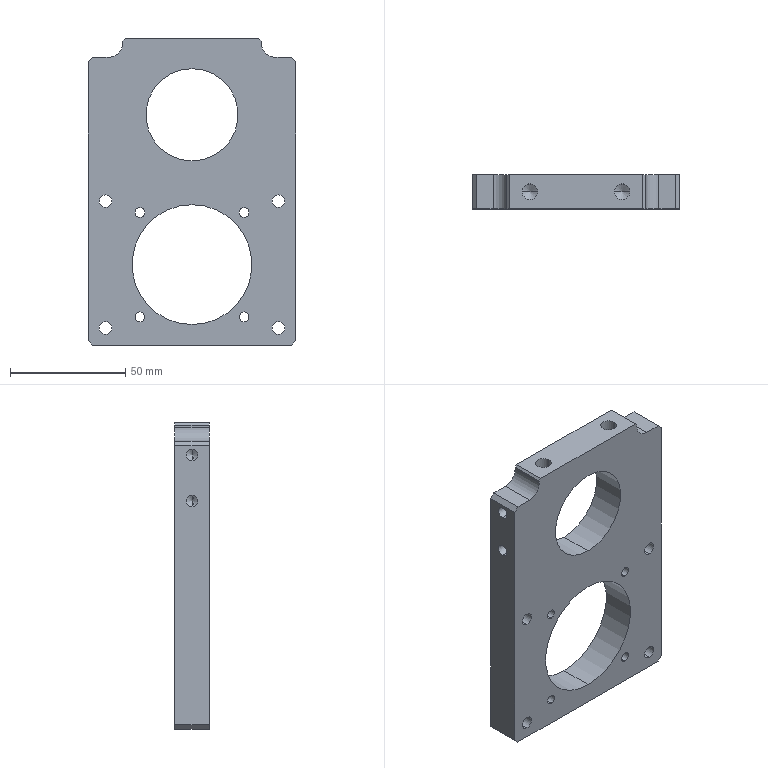Component | SolidWorks | H2020022-0413-1-1 | 1 solid | 74 faces | box 90 x 14.8 x 133 mm | volume 117995 mm3 | cylinder 42 | plane 20 | cone 12 | commonest cylinder face diameters 5 x8 4.2 x8 10 x8 5.5 x8 6.8 x4 40 x2 52 x2 12 x2 | material 6061 Aluminum Alloy
build123d program:
from build123d import *

# Parameters (mm, degrees)
SKETCH1_W                                       = 90
SKETCH1_H                                       = 125
BOSS_EXTRUDE1_DEPTH                             = 14.8
SKETCH4_R                                       = 26
CUT_EXTRUDE1_DEPTH                              = 155.739
M5_HEX_SOCKET_HEAD_CAP_SCREW_CBORE1_D           = 5.5
M5_HEX_SOCKET_HEAD_CAP_SCREW_CBORE1_CBORE_D     = 10
M5_HEX_SOCKET_HEAD_CAP_SCREW_CBORE1_CBORE_DEPTH = 5.4
M6_TAPPED_HOLE1_AT_2_COUNT                      = 2
M6_TAPPED_HOLE1_AT_2_PITCH                      = 20
CHAMFER1_SIZE                                   = 2
M5_TAPPED_HOLE2_D                               = 4.2
CIRPATTERN1_COUNT                               = 4
SKETCH20_R                                      = 20
CUT_EXTRUDE4_DEPTH                              = 155.739
SKETCH21_W                                      = 8
SKETCH21_H                                      = 14.8
BOSS_EXTRUDE2_DEPTH                             = 30
M8_TAPPED_HOLE1_D                               = 6.8
M8_TAPPED_HOLE1_DEPTH                           = 13.75
M8_TAPPED_HOLE1_TIP                             = 2.043
FILLET1_R                                       = 6
CHAMFER2_SIZE                                   = 1


with BuildPart() as part:
    # Sketch1 → Boss-Extrude1 (new body)
    with BuildSketch(Plane(origin=(0, 0, 0), x_dir=(1, 0, 0), z_dir=(0, 1, 0))):
        with Locations((45, 62.5)):
            Rectangle(SKETCH1_W, SKETCH1_H)
    extrude(amount=BOSS_EXTRUDE1_DEPTH)

    # Sketch4 → Cut-Extrude1 (cut, through all)
    with BuildSketch(Plane(origin=(0, 14.8, 0), x_dir=(1, 0, 0), z_dir=(0, 1, 0))):
        with Locations(Location((45, 90, 0), (0, 0, 270))):
            Circle(SKETCH4_R)
    extrude(amount=-CUT_EXTRUDE1_DEPTH, mode=Mode.SUBTRACT)

    # M5 Hex Socket Head Cap Screw CBORE1 (through all)
    with Locations(Plane(origin=(0, 14.8, 0), x_dir=(1, 0, 0), z_dir=(0, 1, 0))):
        with Locations((7.5, 62.5), (82.5, 62.5), (82.5, 117.5), (7.5, 117.5)):
            CounterBoreHole(M5_HEX_SOCKET_HEAD_CAP_SCREW_CBORE1_D / 2, M5_HEX_SOCKET_HEAD_CAP_SCREW_CBORE1_CBORE_D / 2, M5_HEX_SOCKET_HEAD_CAP_SCREW_CBORE1_CBORE_DEPTH)

    # Sketch12 → M6 Tapped Hole1 (revolve, cut)
    with BuildSketch(Plane(origin=(90, 7.4, -6), x_dir=(0, 0, -1), z_dir=(0, 1, 0))):
        Polygon((0, 0), (0, 16.502), (2.5, 15), (2.5, 0), align=None)
    m6_tapped_hole1 = revolve(axis=Axis((96.35, 7.4, -6), (-1, 0, 0)), mode=Mode.SUBTRACT)

    # M6 Tapped Hole1 at 2: M6 Tapped Hole1 ×2
    with Locations(*[(0, 0, -i * M6_TAPPED_HOLE1_AT_2_PITCH) for i in range(1, M6_TAPPED_HOLE1_AT_2_COUNT)]):
        add(m6_tapped_hole1, mode=Mode.SUBTRACT)

    # Chamfer1
    chamfer1_edges = [part.edges().sort_by_distance(p)[0] for p in [
        (0, 7.4, -125),
        (90, 7.4, -125),
        (90, 7.4, 0),
        (0, 7.4, 0),
    ]]
    chamfer(chamfer1_edges, length=CHAMFER1_SIZE)

    # M5 Tapped Hole2 (through all)
    with Locations(Plane(origin=(0, 14.8, 0), x_dir=(1, 0, 0), z_dir=(0, 1, 0))):
        with Locations((22.373, 112.627)):
            m5_tapped_hole2 = Hole(M5_TAPPED_HOLE2_D / 2)

    # CirPattern1: M5 Tapped Hole2 ×4 about axis
    cirpattern1_axis = Axis((45, 0, -90), (0, 1, 0))
    for i in range(1, CIRPATTERN1_COUNT):
        add(m5_tapped_hole2.rotate(cirpattern1_axis, i * 360 / CIRPATTERN1_COUNT), mode=Mode.SUBTRACT)

    # Sketch20 → Cut-Extrude4 (cut, through all)
    with BuildSketch(Plane(origin=(0, 14.8, 0), x_dir=(1, 0, 0), z_dir=(0, 1, 0))):
        with Locations(Location((45, 25, 0), (0, 0, 270))):
            Circle(SKETCH20_R)
    extrude(amount=-CUT_EXTRUDE4_DEPTH, mode=Mode.SUBTRACT)

    # Sketch21 → Boss-Extrude2 (add, symmetric)
    with BuildSketch(Plane(origin=(45, 0, 0), x_dir=(0, 0, -1), z_dir=(1, 0, 0))):
        with Locations((-4, 7.4)):
            Rectangle(SKETCH21_W, SKETCH21_H)
    extrude(amount=BOSS_EXTRUDE2_DEPTH, both=True)

    # M8 Tapped Hole1
    with Locations(Plane.XY.offset(8)):
        with Locations((25, 7.4), (65, 7.4)):
            Hole(M8_TAPPED_HOLE1_D / 2, depth=M8_TAPPED_HOLE1_DEPTH)
            with Locations((0, 0, -(M8_TAPPED_HOLE1_DEPTH + M8_TAPPED_HOLE1_TIP / 2))):  # 118° drill point
                Cone(0, M8_TAPPED_HOLE1_D / 2, M8_TAPPED_HOLE1_TIP, mode=Mode.SUBTRACT)

    # Fillet1
    fillet1_edges = [part.edges().sort_by_distance(p)[0] for p in [
        (15, 7.4, 0),
        (75, 7.4, 0),
    ]]
    fillet(fillet1_edges, radius=FILLET1_R)

    # Chamfer2
    chamfer2_edges = [part.edges().sort_by_distance(p)[0] for p in [
        (15, 7.4, 8),
        (75, 7.4, 8),
    ]]
    chamfer(chamfer2_edges, length=CHAMFER2_SIZE)

    # Mirror1: M6 Tapped Hole1 across plane
    add(m6_tapped_hole1.mirror(Plane.ZY.offset(-45)), mode=Mode.SUBTRACT)

    # Mirror1 copy 1 sketch → Mirror1 copy 1 (revolve, cut)
    with BuildSketch(Plane(origin=(0, 7.4, -26), x_dir=(0, 0, -1), z_dir=(0, 1, 0))):
        Polygon((0, 0), (0, -16.502), (2.5, -15), (2.5, 0), align=None)
    revolve(axis=Axis((-6.35, 7.4, -26), (-1, 0, 0)), mode=Mode.SUBTRACT)


solid = part.part

# Placed as in the assembly
solid = solid.moved(Location((-75.964, 102.013, 370.197), (0, 0, 0)))